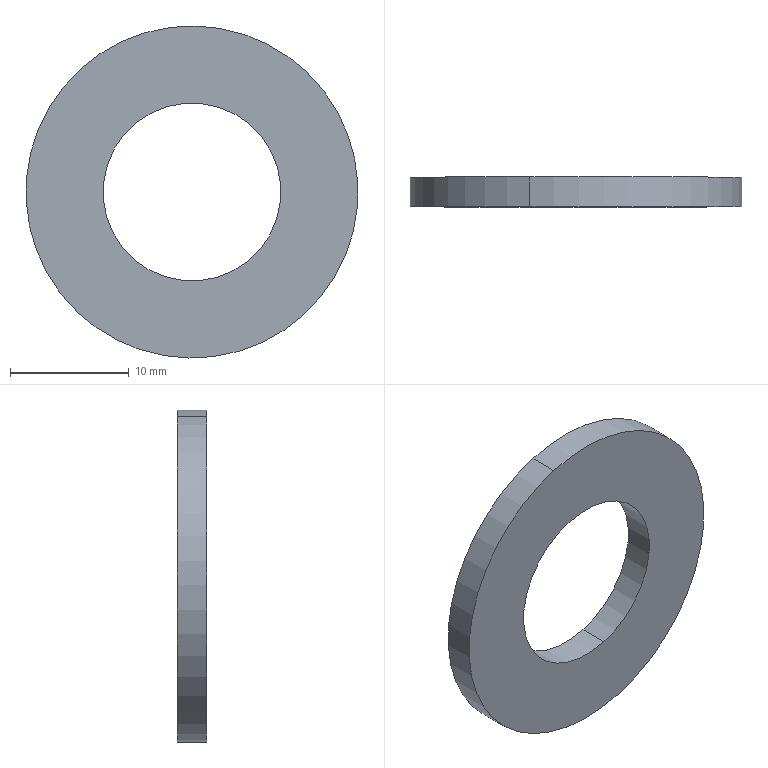Component | SolidWorks | 24FlatWasher_GradeA[GBT97_1-2002][14]-1 | 1 solid | 6 faces | box 28 x 2.5 x 28 mm | volume 1098 mm3 | cylinder 4 | plane 2 | commonest cylinder face diameters 28 x2 15 x2 | material Alloy Steel
build123d program:
from build123d import *

# Parameters (mm, degrees)
SKETCH1_W = 6.5
SKETCH1_H = 2.5


with BuildPart() as part:
    # Sketch1 → Matrix-Rotate1 (revolve)
    with BuildSketch(Plane.XY, mode=Mode.PRIVATE) as matrix_rotate1_sk:
        with Locations((-10.75, 9.895)):
            Rectangle(SKETCH1_W, SKETCH1_H)
    revolve(matrix_rotate1_sk.sketch.rotate(Axis((0, 0, 0), (0, 1, 0)), 270), axis=Axis((0, 0, 0), (0, 1, 0)))


solid = part.part

# Placed as in the assembly
solid = solid.moved(Location((-35.115, 82.664, 610), (0, 0, 0)))
STEP:
#1=CARTESIAN_POINT('',(-1.535,3.693,24.545));
#2=VERTEX_POINT('',#1);
#3=CARTESIAN_POINT('',(-1.23,3.693,23.486));
#4=VERTEX_POINT('',#3);
#5=CARTESIAN_POINT('',(-1.382,3.693,24.016));
#6=DIRECTION('',(0.,-1.,0.));
#7=DIRECTION('',(-0.2774,0.,0.9608));
#8=AXIS2_PLACEMENT_3D('',#5,#6,#7);
#9=CIRCLE('',#8,0.5512);
#10=EDGE_CURVE('',#2,#4,#9,.T.);
#11=ORIENTED_EDGE('',*,*,#10,.T.);
#12=CARTESIAN_POINT('',(-1.23,3.595,23.486));
#13=VERTEX_POINT('',#12);
#14=CARTESIAN_POINT('',(-1.23,3.255,23.486));
#15=DIRECTION('',(0.,-1.,0.));
#16=VECTOR('',#15,39.37);
#17=LINE('',#14,#16);
#18=EDGE_CURVE('',#4,#13,#17,.T.);
#19=ORIENTED_EDGE('',*,*,#18,.T.);
#20=CARTESIAN_POINT('',(-1.535,3.595,24.545));
#21=VERTEX_POINT('',#20);
#22=CARTESIAN_POINT('',(-1.382,3.595,24.016));
#23=DIRECTION('',(0.,-1.,0.));
#24=DIRECTION('',(-0.2774,0.,0.9608));
#25=AXIS2_PLACEMENT_3D('',#22,#23,#24);
#26=CIRCLE('',#25,0.5512);
#27=EDGE_CURVE('',#21,#13,#26,.T.);
#28=ORIENTED_EDGE('',*,*,#27,.F.);
#29=CARTESIAN_POINT('',(-1.535,3.255,24.545));
#30=DIRECTION('',(0.,-1.,0.));
#31=VECTOR('',#30,39.37);
#32=LINE('',#29,#31);
#33=EDGE_CURVE('',#2,#21,#32,.T.);
#34=ORIENTED_EDGE('',*,*,#33,.F.);
#35=EDGE_LOOP('',(#11,#19,#28,#34));
#36=FACE_OUTER_BOUND('',#35,.T.);
#37=CARTESIAN_POINT('',(-1.382,3.255,24.016));
#38=DIRECTION('',(0.,-1.,0.));
#39=DIRECTION('',(-0.2774,0.,0.9608));
#40=AXIS2_PLACEMENT_3D('',#37,#38,#39);
#41=CYLINDRICAL_SURFACE('',#40,0.5512);
#42=ADVANCED_FACE('',(#36),#41,.T.);
#43=CARTESIAN_POINT('',(-1.301,3.693,23.732));
#44=VERTEX_POINT('',#43);
#45=CARTESIAN_POINT('',(-1.464,3.693,24.299));
#46=VERTEX_POINT('',#45);
#47=CARTESIAN_POINT('',(-1.382,3.693,24.016));
#48=DIRECTION('',(0.,-1.,0.));
#49=DIRECTION('',(-0.2774,0.,0.9608));
#50=AXIS2_PLACEMENT_3D('',#47,#48,#49);
#51=CIRCLE('',#50,0.2953);
#52=EDGE_CURVE('',#44,#46,#51,.T.);
#53=ORIENTED_EDGE('',*,*,#52,.F.);
#54=CARTESIAN_POINT('',(-1.301,3.595,23.732));
#55=VERTEX_POINT('',#54);
#56=CARTESIAN_POINT('',(-1.301,3.255,23.732));
#57=DIRECTION('',(0.,-1.,0.));
#58=VECTOR('',#57,39.37);
#59=LINE('',#56,#58);
#60=EDGE_CURVE('',#44,#55,#59,.T.);
#61=ORIENTED_EDGE('',*,*,#60,.T.);
#62=CARTESIAN_POINT('',(-1.464,3.595,24.299));
#63=VERTEX_POINT('',#62);
#64=CARTESIAN_POINT('',(-1.382,3.595,24.016));
#65=DIRECTION('',(0.,-1.,0.));
#66=DIRECTION('',(-0.2774,0.,0.9608));
#67=AXIS2_PLACEMENT_3D('',#64,#65,#66);
#68=CIRCLE('',#67,0.2953);
#69=EDGE_CURVE('',#55,#63,#68,.T.);
#70=ORIENTED_EDGE('',*,*,#69,.T.);
#71=CARTESIAN_POINT('',(-1.464,3.255,24.299));
#72=DIRECTION('',(0.,-1.,0.));
#73=VECTOR('',#72,39.37);
#74=LINE('',#71,#73);
#75=EDGE_CURVE('',#46,#63,#74,.T.);
#76=ORIENTED_EDGE('',*,*,#75,.F.);
#77=EDGE_LOOP('',(#53,#61,#70,#76));
#78=FACE_OUTER_BOUND('',#77,.T.);
#79=CARTESIAN_POINT('',(-1.382,3.255,24.016));
#80=DIRECTION('',(0.,-1.,0.));
#81=DIRECTION('',(-0.2774,0.,0.9608));
#82=AXIS2_PLACEMENT_3D('',#79,#80,#81);
#83=CYLINDRICAL_SURFACE('',#82,0.2953);
#84=ADVANCED_FACE('',(#78),#83,.F.);
#85=ORIENTED_EDGE('',*,*,#60,.F.);
#86=CARTESIAN_POINT('',(-1.382,3.693,24.016));
#87=DIRECTION('',(0.,-1.,0.));
#88=DIRECTION('',(-0.2774,0.,0.9608));
#89=AXIS2_PLACEMENT_3D('',#86,#87,#88);
#90=CIRCLE('',#89,0.2953);
#91=EDGE_CURVE('',#46,#44,#90,.T.);
#92=ORIENTED_EDGE('',*,*,#91,.F.);
#93=ORIENTED_EDGE('',*,*,#75,.T.);
#94=CARTESIAN_POINT('',(-1.382,3.595,24.016));
#95=DIRECTION('',(0.,-1.,0.));
#96=DIRECTION('',(-0.2774,0.,0.9608));
#97=AXIS2_PLACEMENT_3D('',#94,#95,#96);
#98=CIRCLE('',#97,0.2953);
#99=EDGE_CURVE('',#63,#55,#98,.T.);
#100=ORIENTED_EDGE('',*,*,#99,.T.);
#101=EDGE_LOOP('',(#85,#92,#93,#100));
#102=FACE_OUTER_BOUND('',#101,.T.);
#103=CARTESIAN_POINT('',(-1.382,3.255,24.016));
#104=DIRECTION('',(0.,-1.,0.));
#105=DIRECTION('',(-0.2774,0.,0.9608));
#106=AXIS2_PLACEMENT_3D('',#103,#104,#105);
#107=CYLINDRICAL_SURFACE('',#106,0.2953);
#108=ADVANCED_FACE('',(#102),#107,.F.);
#109=ORIENTED_EDGE('',*,*,#10,.F.);
#110=CARTESIAN_POINT('',(-1.382,3.693,24.016));
#111=DIRECTION('',(0.,-1.,0.));
#112=DIRECTION('',(-0.2774,0.,0.9608));
#113=AXIS2_PLACEMENT_3D('',#110,#111,#112);
#114=CIRCLE('',#113,0.5512);
#115=EDGE_CURVE('',#4,#2,#114,.T.);
#116=ORIENTED_EDGE('',*,*,#115,.F.);
#117=EDGE_LOOP('',(#109,#116));
#118=FACE_OUTER_BOUND('',#117,.T.);
#119=ORIENTED_EDGE('',*,*,#91,.T.);
#120=ORIENTED_EDGE('',*,*,#52,.T.);
#121=EDGE_LOOP('',(#119,#120));
#122=FACE_BOUND('',#121,.T.);
#123=CARTESIAN_POINT('',(-1.099,3.693,24.098));
#124=DIRECTION('',(0.,-1.,0.));
#125=DIRECTION('',(-0.2774,0.,0.9608));
#126=AXIS2_PLACEMENT_3D('',#123,#124,#125);
#127=PLANE('',#126);
#128=ADVANCED_FACE('',(#118,#122),#127,.F.);
#129=ORIENTED_EDGE('',*,*,#18,.F.);
#130=ORIENTED_EDGE('',*,*,#115,.T.);
#131=ORIENTED_EDGE('',*,*,#33,.T.);
#132=CARTESIAN_POINT('',(-1.382,3.595,24.016));
#133=DIRECTION('',(0.,-1.,0.));
#134=DIRECTION('',(-0.2774,0.,0.9608));
#135=AXIS2_PLACEMENT_3D('',#132,#133,#134);
#136=CIRCLE('',#135,0.5512);
#137=EDGE_CURVE('',#13,#21,#136,.T.);
#138=ORIENTED_EDGE('',*,*,#137,.F.);
#139=EDGE_LOOP('',(#129,#130,#131,#138));
#140=FACE_OUTER_BOUND('',#139,.T.);
#141=CARTESIAN_POINT('',(-1.382,3.255,24.016));
#142=DIRECTION('',(0.,-1.,0.));
#143=DIRECTION('',(-0.2774,0.,0.9608));
#144=AXIS2_PLACEMENT_3D('',#141,#142,#143);
#145=CYLINDRICAL_SURFACE('',#144,0.5512);
#146=ADVANCED_FACE('',(#140),#145,.T.);
#147=ORIENTED_EDGE('',*,*,#99,.F.);
#148=ORIENTED_EDGE('',*,*,#69,.F.);
#149=EDGE_LOOP('',(#147,#148));
#150=FACE_BOUND('',#149,.T.);
#151=ORIENTED_EDGE('',*,*,#27,.T.);
#152=ORIENTED_EDGE('',*,*,#137,.T.);
#153=EDGE_LOOP('',(#151,#152));
#154=FACE_OUTER_BOUND('',#153,.T.);
#155=CARTESIAN_POINT('',(-1.099,3.595,24.098));
#156=DIRECTION('',(0.,1.,0.));
#157=DIRECTION('',(0.2774,0.,-0.9608));
#158=AXIS2_PLACEMENT_3D('',#155,#156,#157);
#159=PLANE('',#158);
#160=ADVANCED_FACE('',(#150,#154),#159,.F.);
#161=CLOSED_SHELL('',(#42,#84,#108,#128,#146,#160));
#162=MANIFOLD_SOLID_BREP('',#161);
#163=CARTESIAN_POINT('',(0.,0.,0.));
#164=DIRECTION('',(0.,0.,1.));
#165=DIRECTION('',(1.,0.,0.));
#166=AXIS2_PLACEMENT_3D('',#163,#164,#165);
#167=(LENGTH_UNIT()NAMED_UNIT(*)SI_UNIT($,.METRE.));
#168=LENGTH_MEASURE_WITH_UNIT(LENGTH_MEASURE(0.0254),#167);
#169=DIMENSIONAL_EXPONENTS(1.,0.,0.,0.,0.,0.,0.);
#170=(CONVERSION_BASED_UNIT('',#168)LENGTH_UNIT()NAMED_UNIT(#169));
#171=UNCERTAINTY_MEASURE_WITH_UNIT(LENGTH_MEASURE(0.00001),#170,'','');
#172=(NAMED_UNIT(*)PLANE_ANGLE_UNIT()SI_UNIT($,.RADIAN.));
#173=(NAMED_UNIT(*)SI_UNIT($,.STERADIAN.)SOLID_ANGLE_UNIT());
#174=(GEOMETRIC_REPRESENTATION_CONTEXT(3)GLOBAL_UNCERTAINTY_ASSIGNED_CONTEXT((#171))GLOBAL_UNIT_ASSIGNED_CONTEXT((#170,#172,#173))REPRESENTATION_CONTEXT('',''));
#175=ADVANCED_BREP_SHAPE_REPRESENTATION('',(#162,#166),#174);
#176=COLOUR_RGB('',0.7922,0.8196,0.9333);
#177=FILL_AREA_STYLE_COLOUR('',#176);
#178=FILL_AREA_STYLE('',(#177));
#179=SURFACE_STYLE_FILL_AREA(#178);
#180=SURFACE_SIDE_STYLE('',(#179));
#181=SURFACE_STYLE_USAGE(.BOTH.,#180);
#182=PRESENTATION_STYLE_ASSIGNMENT((#181));
#183=STYLED_ITEM('',(#182),#162);
#184=PRESENTATION_LAYER_ASSIGNMENT('','',(#183));
#185=(LENGTH_UNIT()NAMED_UNIT(*)SI_UNIT($,.METRE.));
#186=LENGTH_MEASURE_WITH_UNIT(LENGTH_MEASURE(0.0254),#185);
#187=DIMENSIONAL_EXPONENTS(1.,0.,0.,0.,0.,0.,0.);
#188=(CONVERSION_BASED_UNIT('',#186)LENGTH_UNIT()NAMED_UNIT(#187));
#189=UNCERTAINTY_MEASURE_WITH_UNIT(LENGTH_MEASURE(0.00001),#188,'','');
#190=(NAMED_UNIT(*)PLANE_ANGLE_UNIT()SI_UNIT($,.RADIAN.));
#191=(NAMED_UNIT(*)SI_UNIT($,.STERADIAN.)SOLID_ANGLE_UNIT());
#192=(GEOMETRIC_REPRESENTATION_CONTEXT(3)GLOBAL_UNCERTAINTY_ASSIGNED_CONTEXT((#189))GLOBAL_UNIT_ASSIGNED_CONTEXT((#188,#190,#191))REPRESENTATION_CONTEXT('',''));
#193=MECHANICAL_DESIGN_GEOMETRIC_PRESENTATION_REPRESENTATION('',(#183),#192);